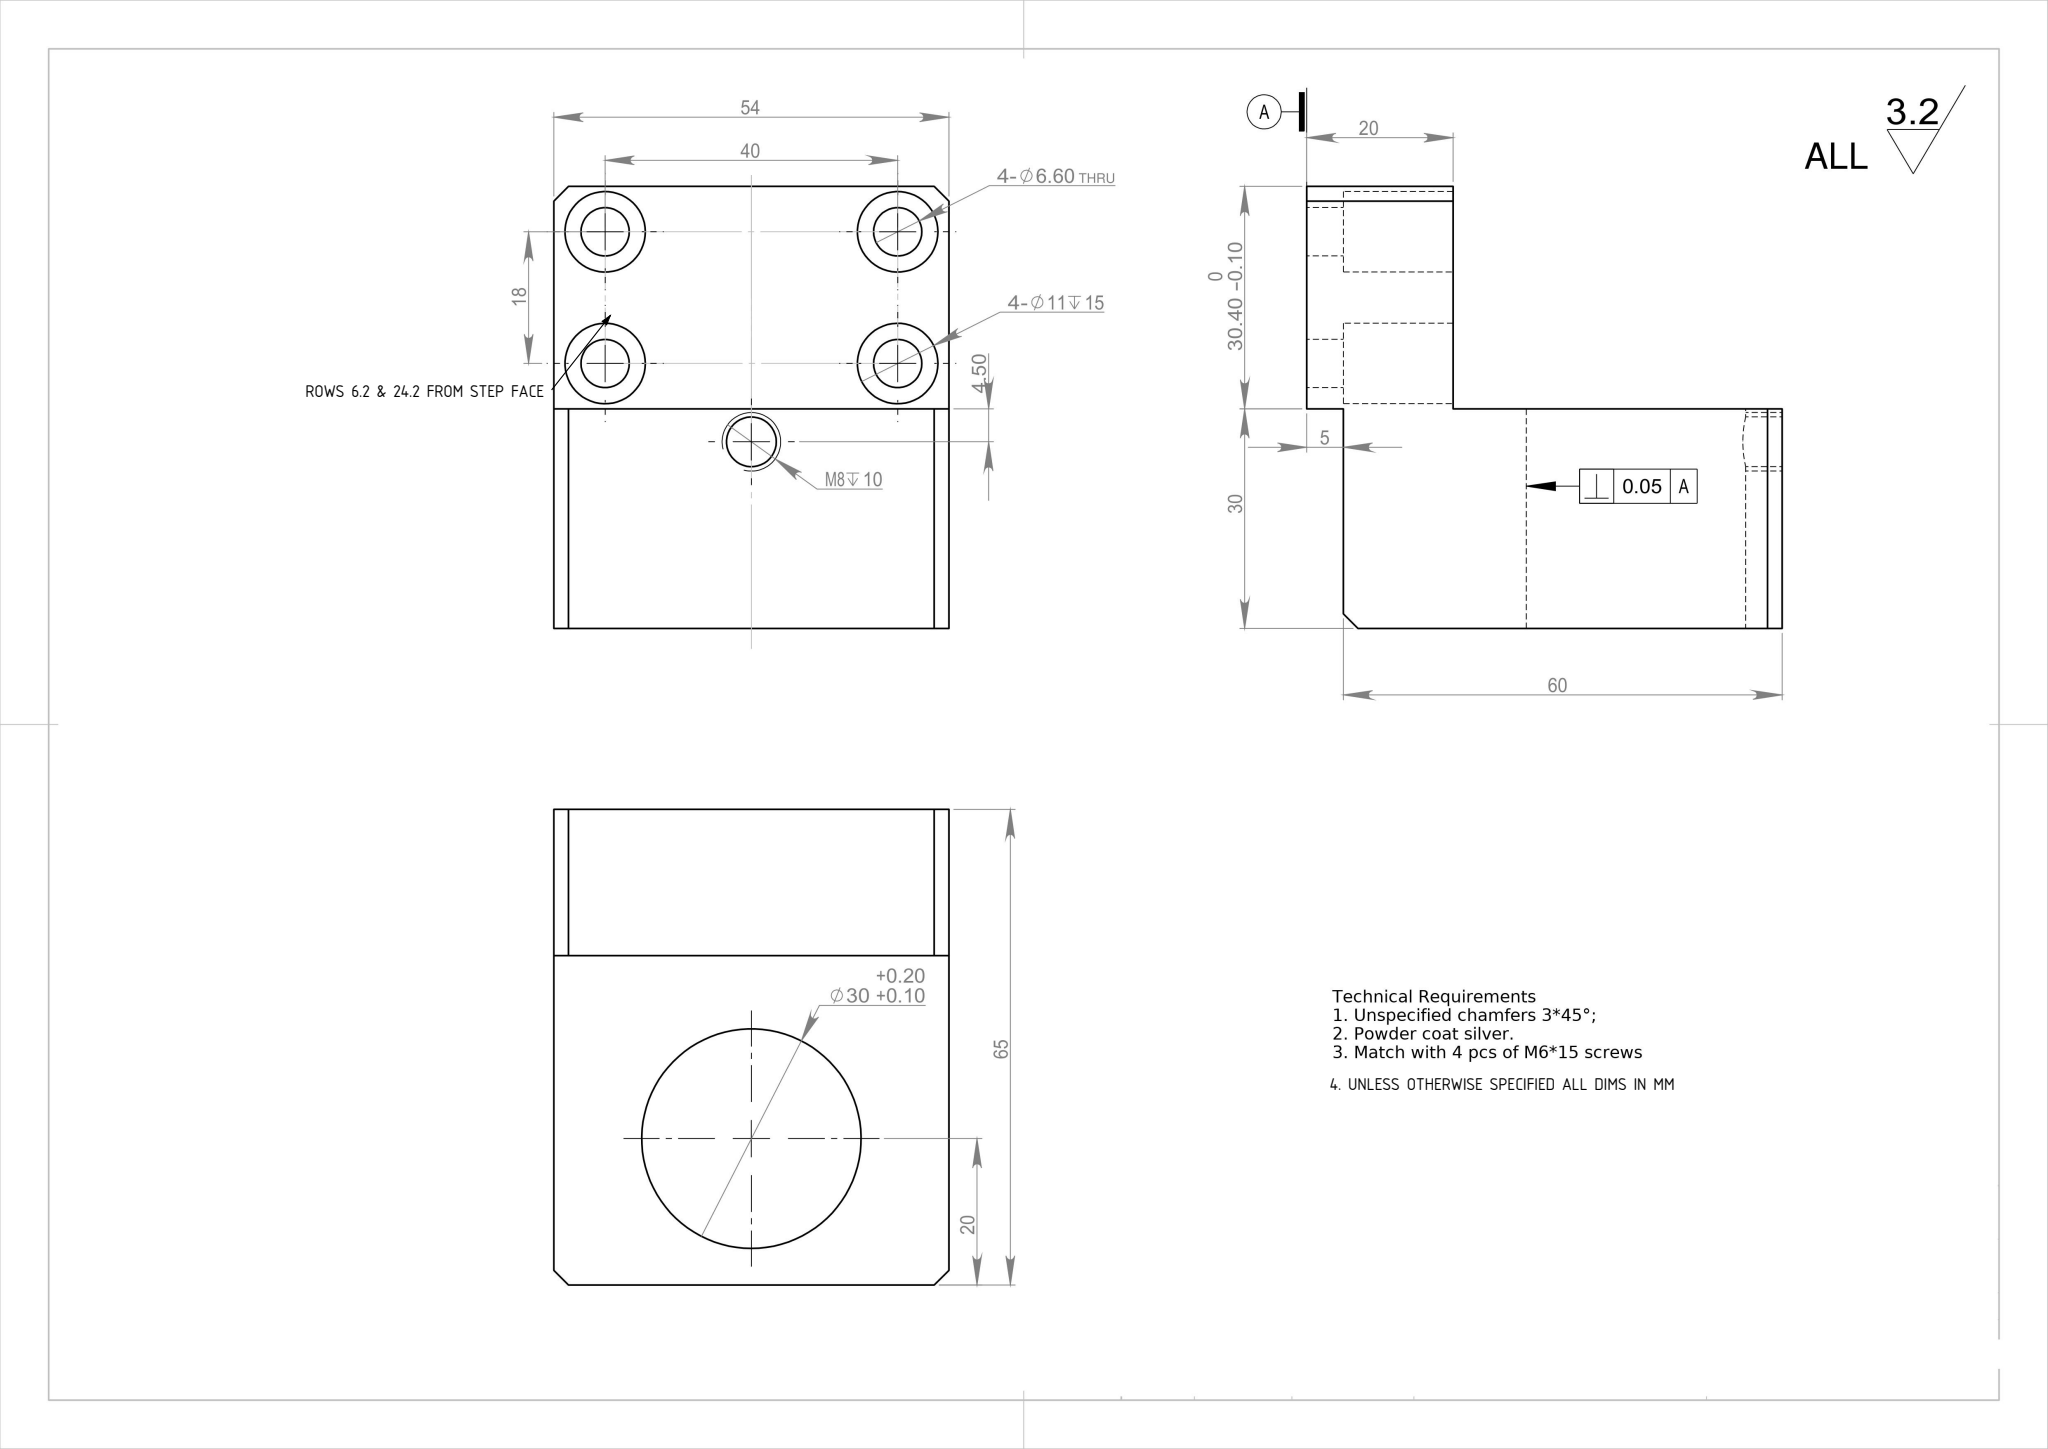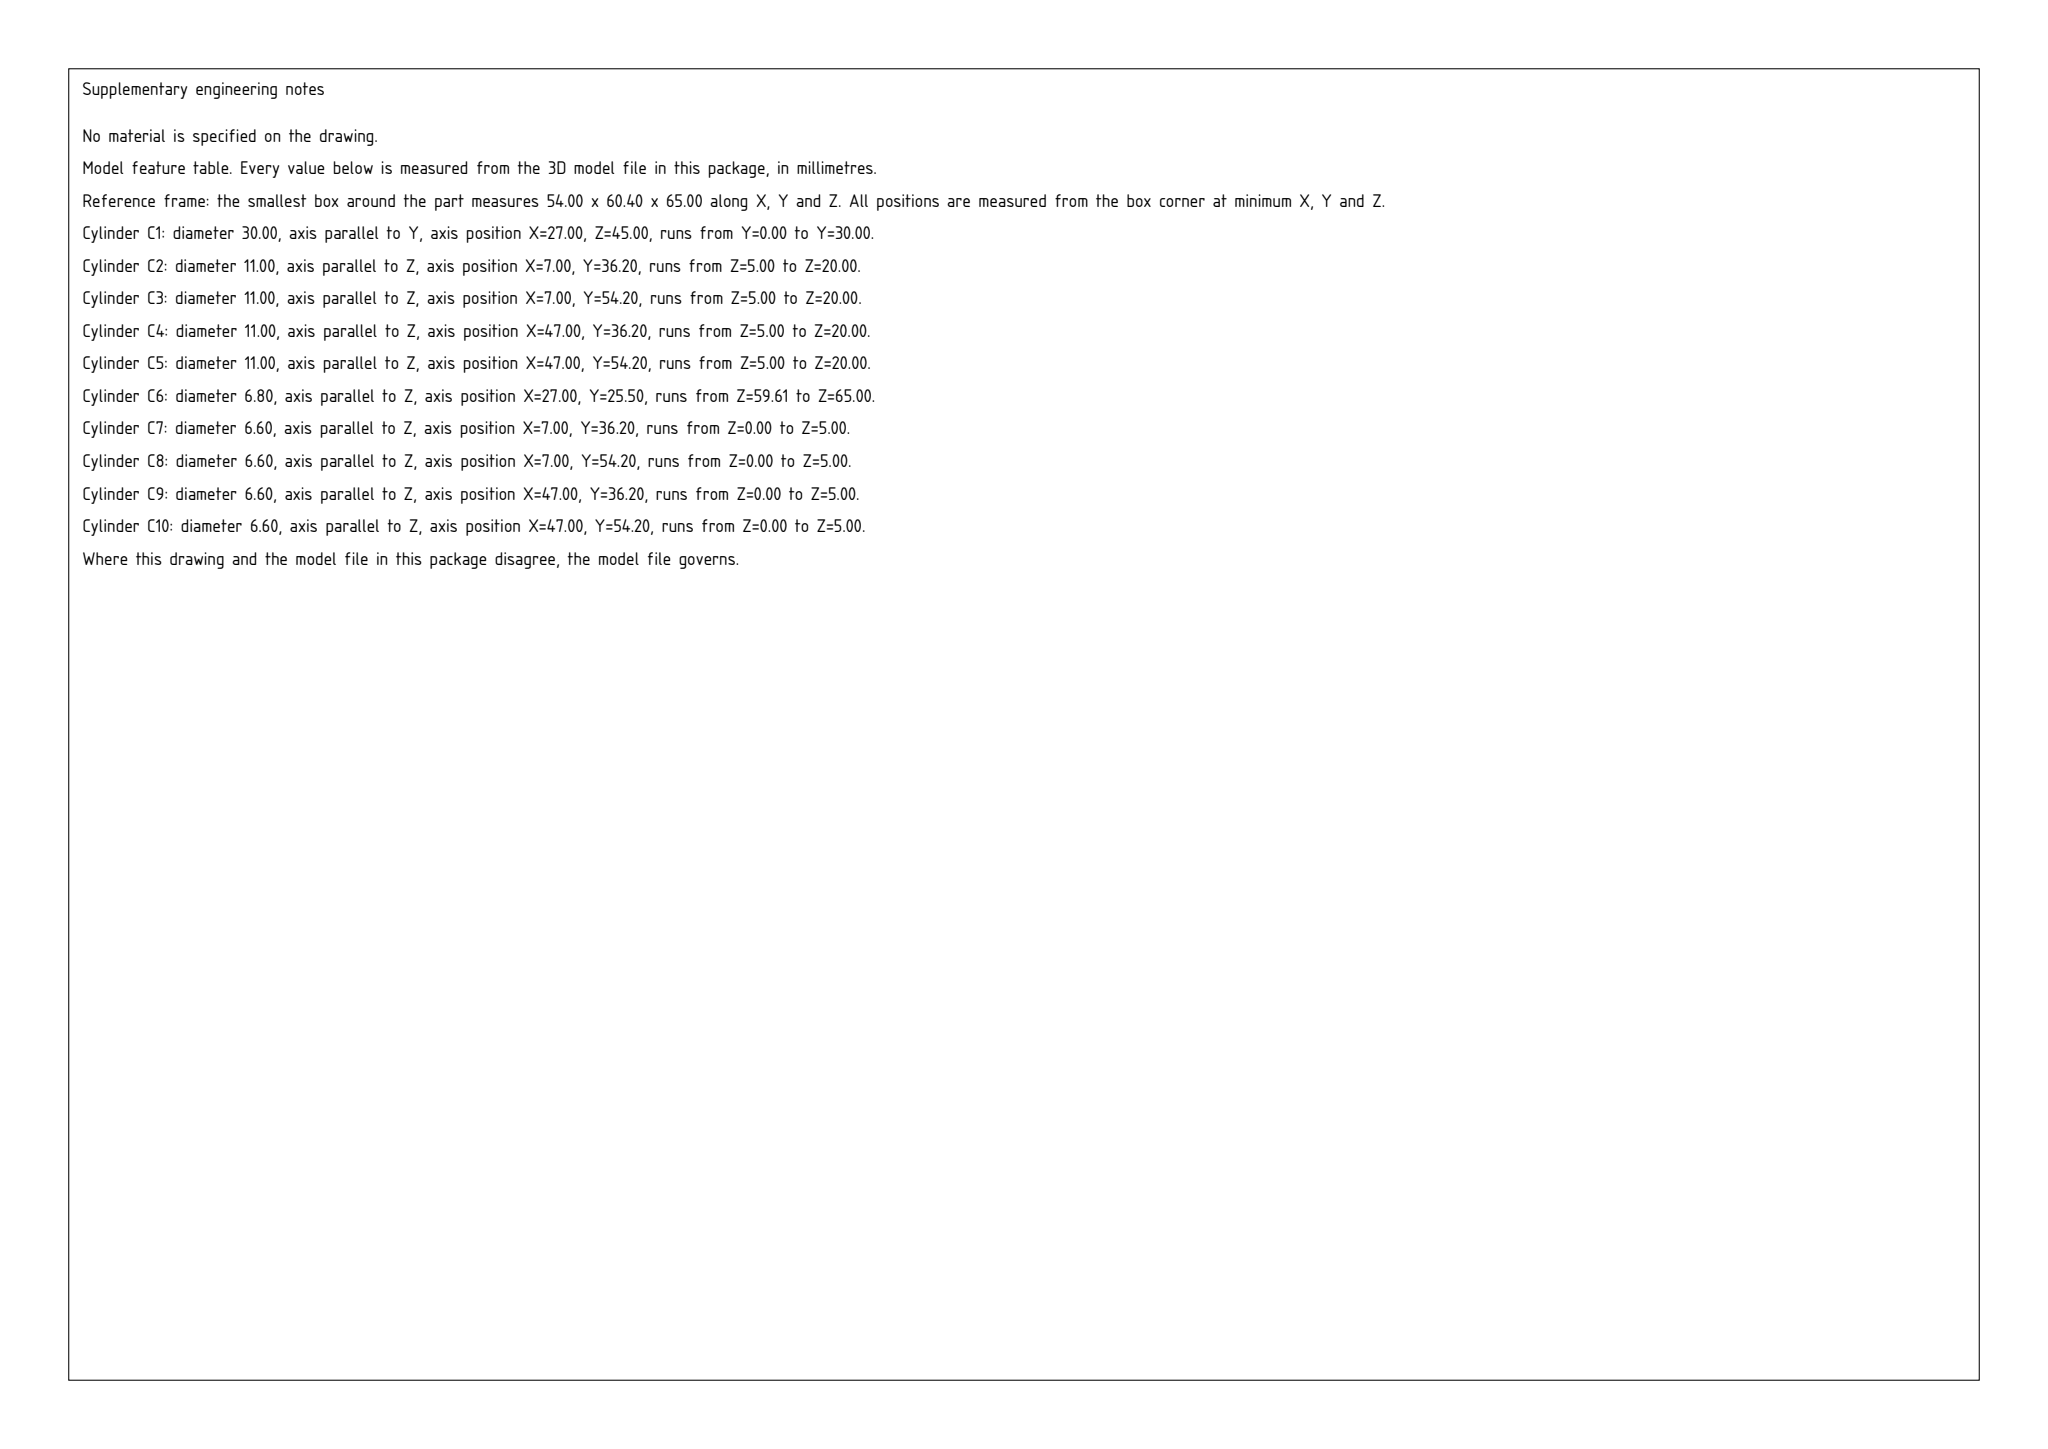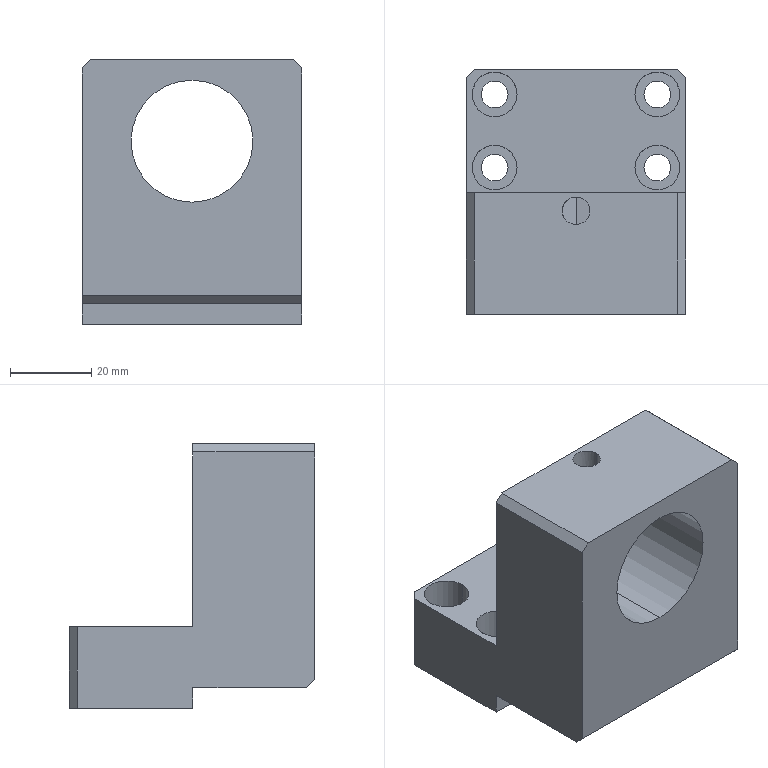Part | SolidWorks | mm | 1 solid | 39 faces | box 54 x 60.4 x 65 mm | volume 101947 mm3 | cylinder 20 | plane 19 | commonest cylinder face diameters 11 x8 6.6 x8 30 x2 6.8 x2
Drawing notes:
FRONT VIEW: C'BORE HOLE ROWS 6.2 & 24.2 FROM STEP FACE | from the solid: Ø6.60/Ø11 axes at y=36.2 & 54.2; step face plane y=30 -> 6.2 and 24.2
UNLESS OTHERWISE SPECIFIED ALL DIMS IN MM | from the solid: STEP model units mm; bbox 54.0 x 60.4 x 65.0 mm
build123d program:
from build123d import *

# Parameters (mm, degrees)
SKETCH1_W                                           = 54
SKETCH1_H                                           = 30
BOSS_EXTRUDE1_DEPTH                                 = 60
M8_TAPPED_HOLE1_D                                   = 6.8
M8_TAPPED_HOLE1_DEPTH                               = 19.75
M8_TAPPED_HOLE1_TIP                                 = 2.043
SKETCH10_W                                          = 54
SKETCH10_H                                          = 15
BOSS_EXTRUDE2_DEPTH                                 = 30.4
SKETCH11_W                                          = 54
SKETCH11_H                                          = 30.4
BOSS_EXTRUDE3_DEPTH                                 = 5
SKETCH3_R                                           = 15
CUT_EXTRUDE4_DEPTH                                  = 73.479
HOLE_SIZE_ACCORDING_TO_TYPE_1_OF_HEXAGO_D           = 6.6
HOLE_SIZE_ACCORDING_TO_TYPE_1_OF_HEXAGO_CBORE_D     = 11
HOLE_SIZE_ACCORDING_TO_TYPE_1_OF_HEXAGO_CBORE_DEPTH = 15
MIRROR6_COPY_1_D                                    = 6.6
MIRROR6_COPY_1_CBORE_D                              = 11
MIRROR6_COPY_1_CBORE_DEPTH                          = 15
CHAMFER1_SIZE                                       = 2


with BuildPart() as part:
    # Sketch1 → Boss-Extrude1 (new body)
    with BuildSketch(Plane.XY):
        Rectangle(SKETCH1_W, SKETCH1_H)
    extrude(amount=BOSS_EXTRUDE1_DEPTH)

    # M8 Tapped Hole1
    with Locations(Plane.XY.offset(60)):
        with Locations((0, 10.5)):
            Hole(M8_TAPPED_HOLE1_D / 2, depth=M8_TAPPED_HOLE1_DEPTH)
            with Locations((0, 0, -(M8_TAPPED_HOLE1_DEPTH + M8_TAPPED_HOLE1_TIP / 2))):  # 118° drill point
                Cone(0, M8_TAPPED_HOLE1_D / 2, M8_TAPPED_HOLE1_TIP, mode=Mode.SUBTRACT)

    # Sketch10 → Boss-Extrude2 (add)
    with BuildSketch(Plane(origin=(0, 15, 0), x_dir=(1, 0, 0), z_dir=(0, 1, 0))):
        with Locations((0, -7.5)):
            Rectangle(SKETCH10_W, SKETCH10_H)
    extrude(amount=BOSS_EXTRUDE2_DEPTH)

    # Sketch11 → Boss-Extrude3 (add)
    with BuildSketch(Plane(origin=(0, 0, 0), x_dir=(-1, 0, 0), z_dir=(0, 0, -1))):
        with Locations((0, 30.2)):
            Rectangle(SKETCH11_W, SKETCH11_H)
    extrude(amount=BOSS_EXTRUDE3_DEPTH)

    # Sketch3 → Cut-Extrude4 (cut, through all)
    with BuildSketch(Plane(origin=(0, 15, 0), x_dir=(1, 0, 0), z_dir=(0, 1, 0))):
        with Locations(Location((0, -40, 0), (0, 0, 270))):
            Circle(SKETCH3_R)
    extrude(amount=-CUT_EXTRUDE4_DEPTH, mode=Mode.SUBTRACT)

    # Hole Size_ according to_Type 1 of Hexago (through all)
    with Locations(Plane.XY.offset(15)):
        with Locations((-20, 39.2)):
            hole_size_according_to_type_1_of_hexago = CounterBoreHole(HOLE_SIZE_ACCORDING_TO_TYPE_1_OF_HEXAGO_D / 2, HOLE_SIZE_ACCORDING_TO_TYPE_1_OF_HEXAGO_CBORE_D / 2, HOLE_SIZE_ACCORDING_TO_TYPE_1_OF_HEXAGO_CBORE_DEPTH)

    # Mirror5: Hole Size_ according to_Type 1 of Hexago across plane
    add(hole_size_according_to_type_1_of_hexago.mirror(Plane(origin=(0, 0, 0), x_dir=(0, 0, 1), z_dir=(1, 0, 0))), mode=Mode.SUBTRACT)

    # Mirror6: Hole Size_ according to_Type 1 of Hexago across plane
    add(hole_size_according_to_type_1_of_hexago.mirror(Plane.ZX.offset(30.2)), mode=Mode.SUBTRACT)

    # Mirror6 copy 1 (through all)
    with Locations(Plane(origin=(0, 60.4, 15), x_dir=(-1, 0, 0), z_dir=(0, 0, 1))):
        with Locations((-20, 39.2)):
            CounterBoreHole(MIRROR6_COPY_1_D / 2, MIRROR6_COPY_1_CBORE_D / 2, MIRROR6_COPY_1_CBORE_DEPTH)

    # Chamfer1
    chamfer1_edges = [part.edges().sort_by_distance(p)[0] for p in [
        (-27, 0, 60),
        (27, 45.4, 5),
        (-27, 45.4, 5),
        (27, 0, 60),
        (0, -15, 0),
    ]]
    chamfer(chamfer1_edges, length=CHAMFER1_SIZE)


solid = part.part